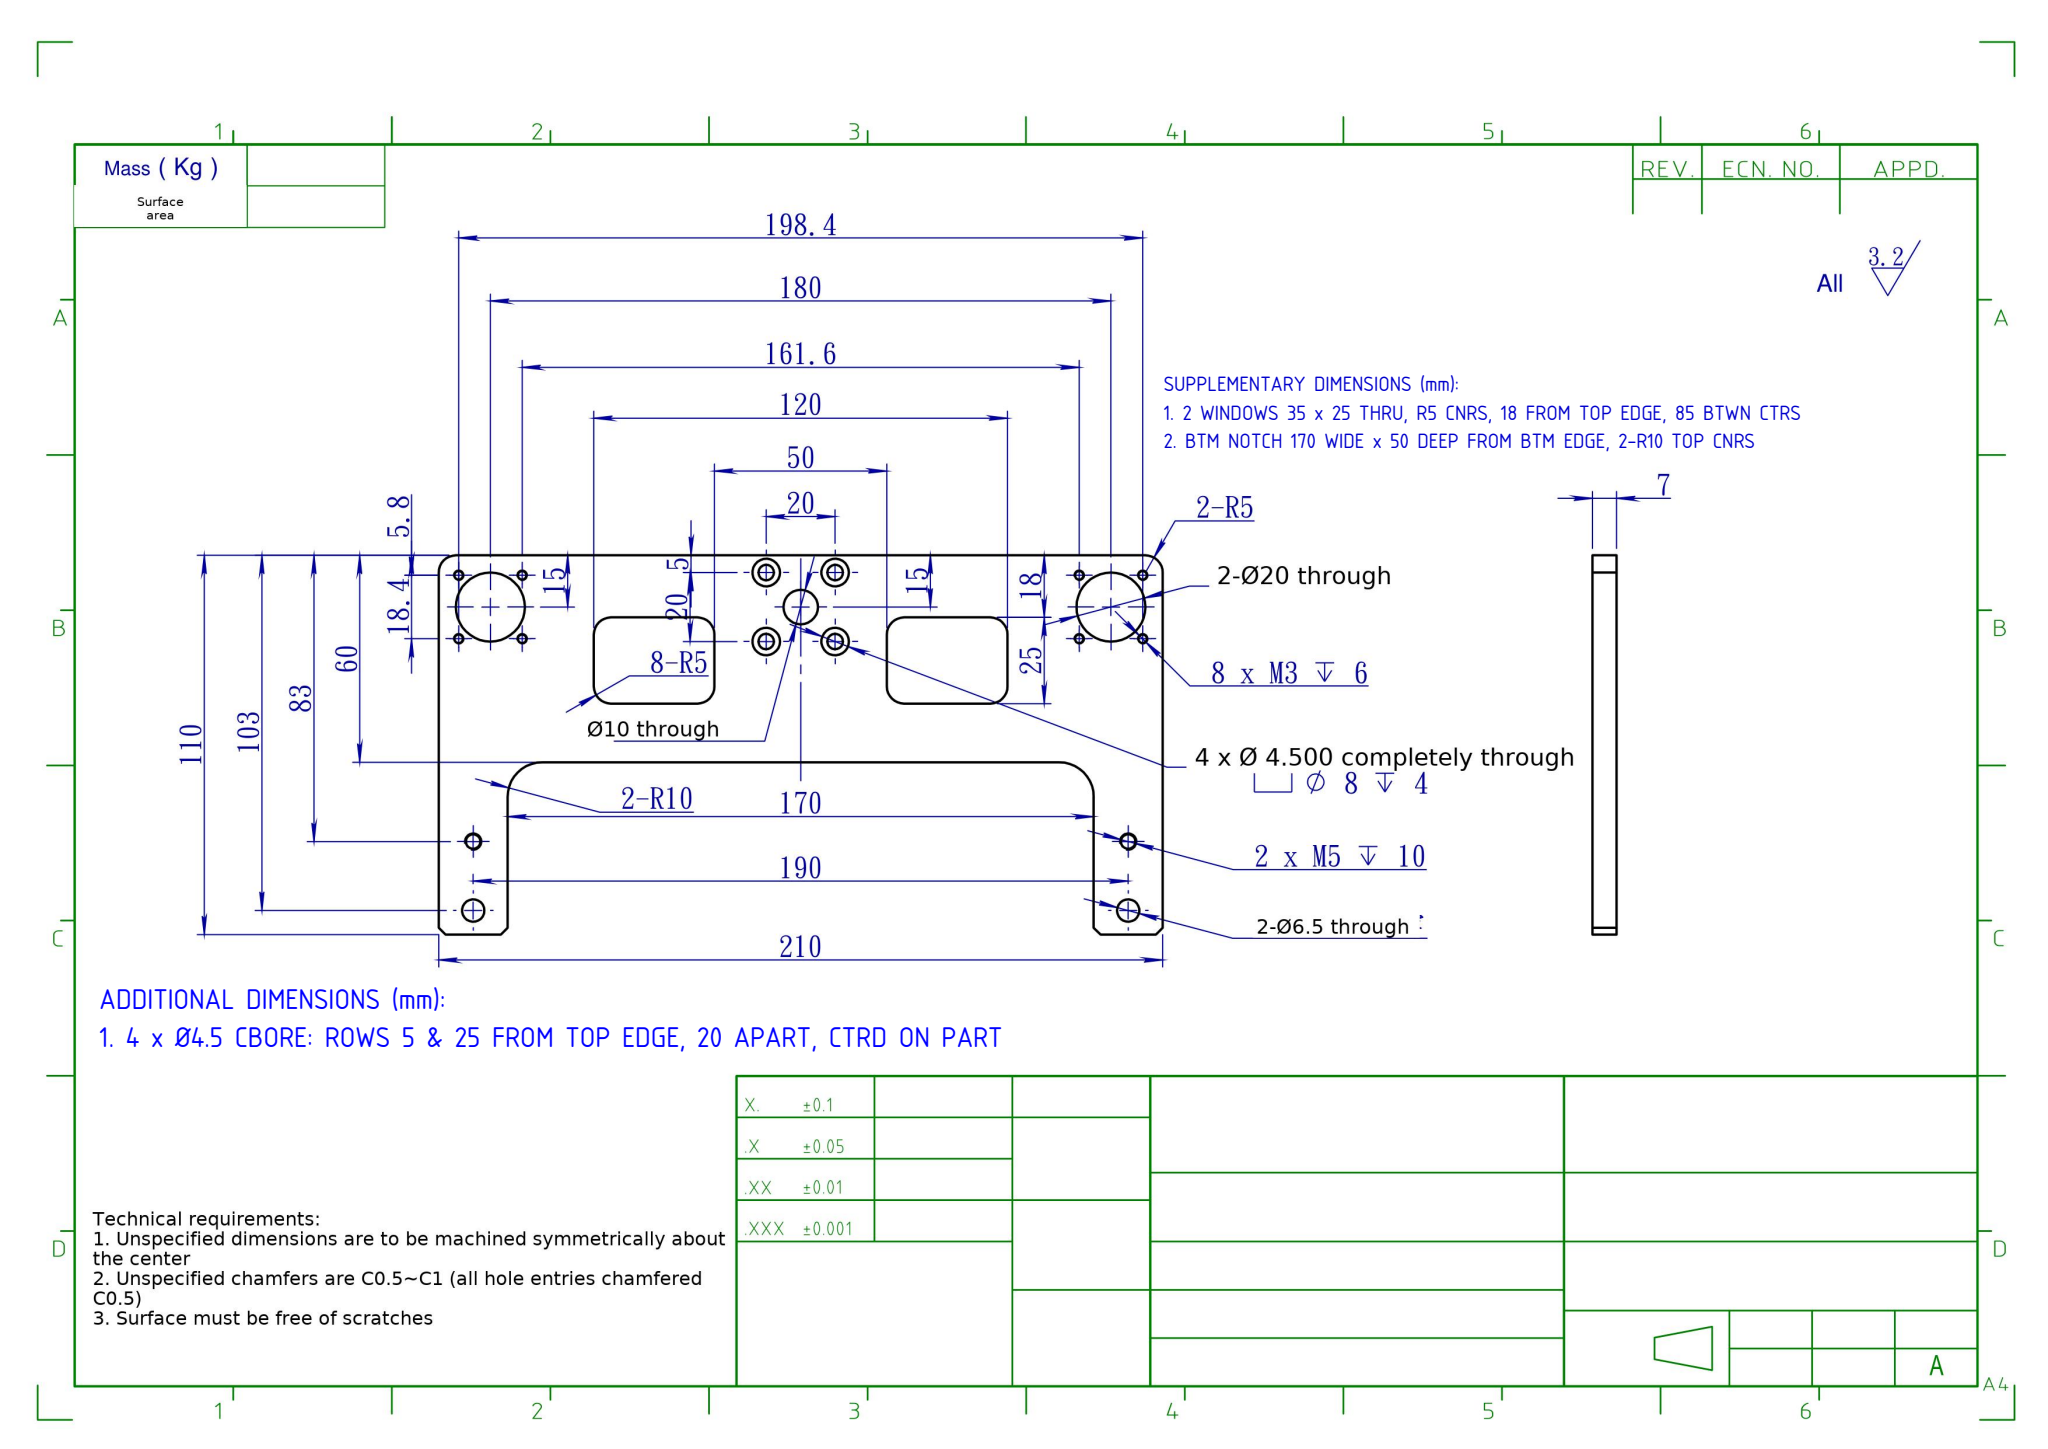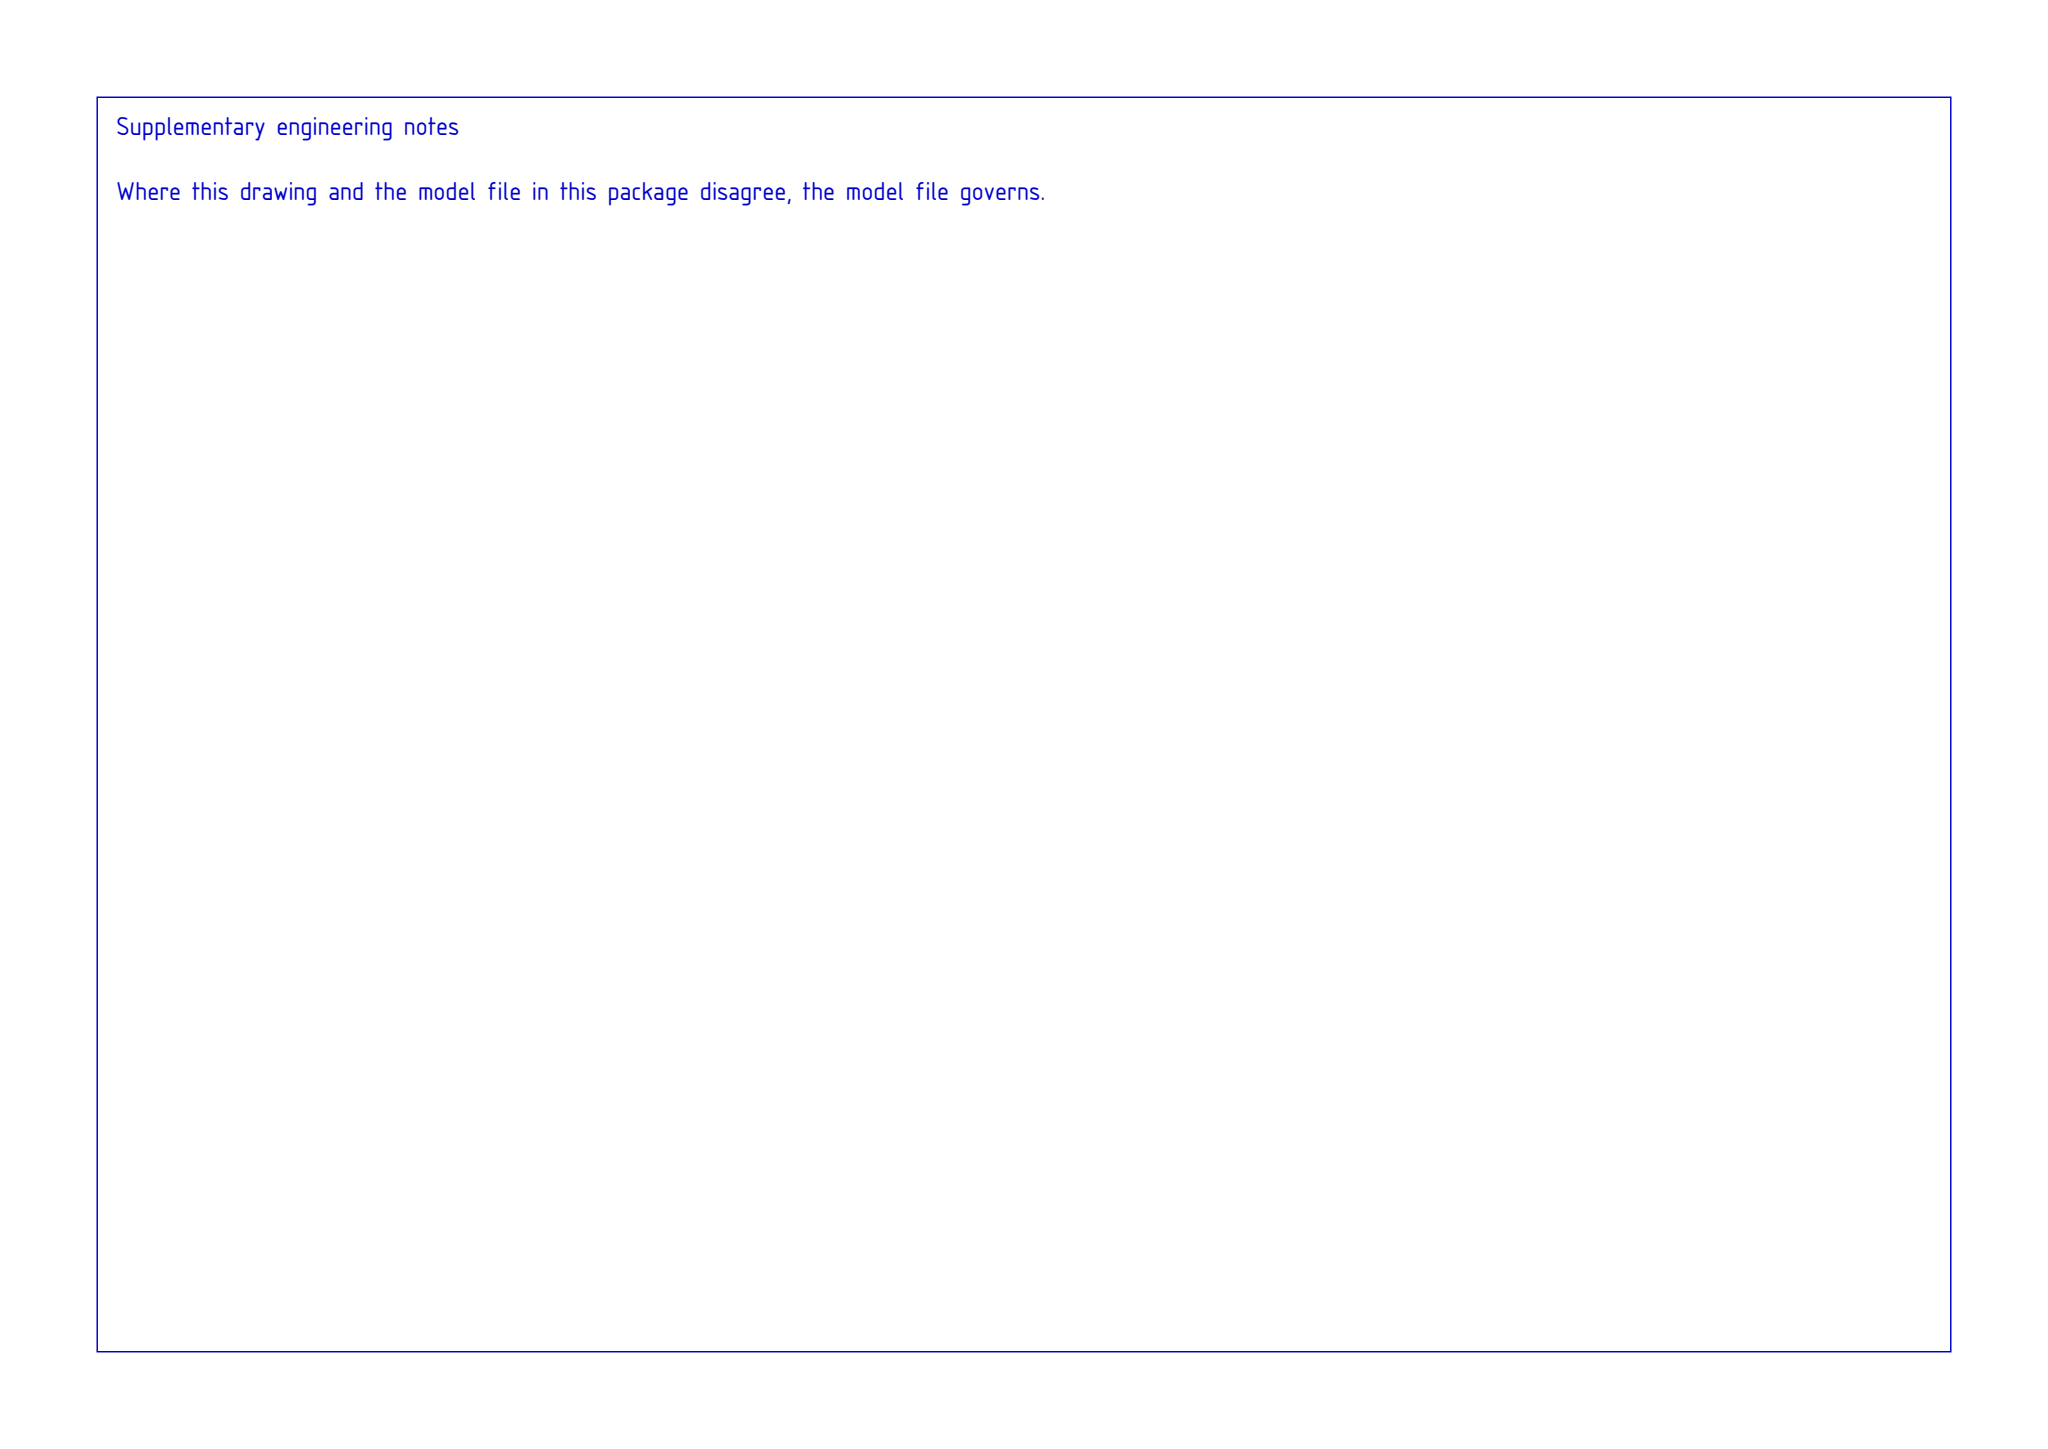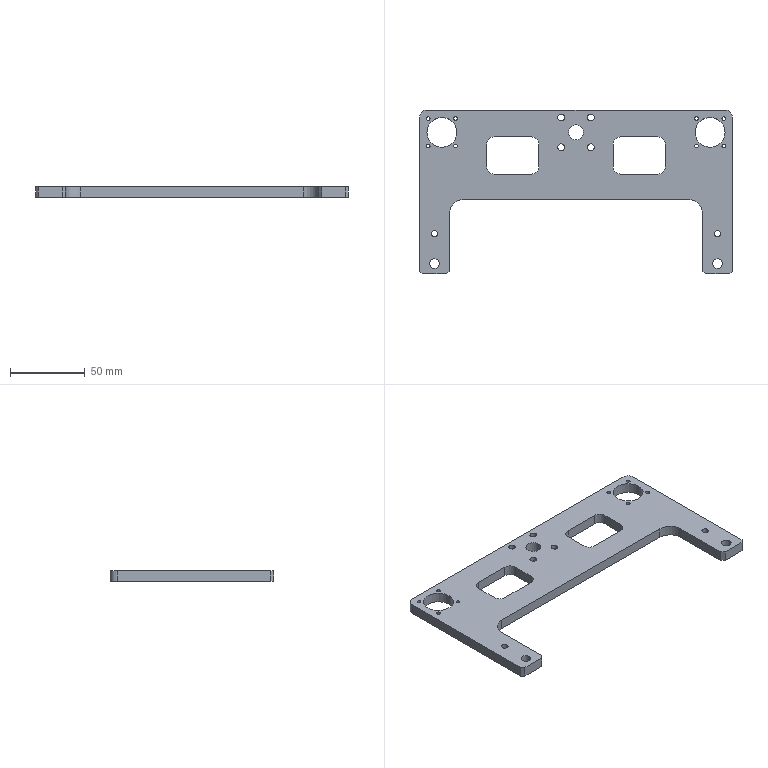Part | SolidWorks | mm | 1 solid | 84 faces | box 210 x 110 x 7 mm | volume 83543 mm3 | cylinder 58 | plane 26 | commonest cylinder face diameters 2.5 x16 10 x12 8 x8 4.5 x8 20 x6 4.2 x4 6.5 x4
build123d program:
from build123d import *

# Parameters (mm, degrees)
SKETCH1_2_W                                         = 210
SKETCH1_2_H                                         = 110
BOSS_EXTRUDE1_DEPTH                                 = 7
SKETCH2_2_W                                         = 170
SKETCH2_2_H                                         = 100
CUT_EXTRUDE1_2_DEPTH                                = 8
FILLET1_R                                           = 10
FILLET2_R                                           = 5
SKETCH3_2_R                                         = 5
SKETCH3_2_R_2                                       = 10
CUT_EXTRUDE2_2_DEPTH                                = 10
SKETCH1_R                                           = 3.25
CUT_EXTRUDE1_DEPTH                                  = 119.739
CHAMFER1_SIZE                                       = 2
M5_TAPPED_HOLE1_D                                   = 4.2
M5_TAPPED_HOLE1_DEPTH                               = 12.4
M5_TAPPED_HOLE1_TIP                                 = 1.262
M3_TAPPED_HOLE1_D                                   = 2.5
M3_TAPPED_HOLE1_DEPTH                               = 7.5
M3_TAPPED_HOLE1_TIP                                 = 0.7511
CBORE_FOR_M4_HEX_SOCKET_HEAD_CAP_SCREW1_D           = 4.5
CBORE_FOR_M4_HEX_SOCKET_HEAD_CAP_SCREW1_CBORE_D     = 8
CBORE_FOR_M4_HEX_SOCKET_HEAD_CAP_SCREW1_CBORE_DEPTH = 4
CUT_EXTRUDE2_DEPTH                                  = 119.739


with BuildPart() as part:
    # Sketch1_2 → Boss-Extrude1 (new body)
    with BuildSketch(Plane.XY):
        Rectangle(SKETCH1_2_W, SKETCH1_2_H)
    extrude(amount=BOSS_EXTRUDE1_DEPTH)

    # Sketch2_2 → Cut-Extrude1_2 (cut)
    with BuildSketch(Plane.XY.offset(7)):
        with Locations((0, -55)):
            Rectangle(SKETCH2_2_W, SKETCH2_2_H)
    extrude(amount=-CUT_EXTRUDE1_2_DEPTH, mode=Mode.SUBTRACT)

    # Fillet1
    fillet1_edges = [part.edges().sort_by_distance(p)[0] for p in [
        (-85, -5, 3.5),
        (85, -5, 3.5),
    ]]
    fillet(fillet1_edges, radius=FILLET1_R)

    # Fillet2
    fillet2_edges = [part.edges().sort_by_distance(p)[0] for p in [
        (-105, 55, 3.5),
        (105, 55, 3.5),
    ]]
    fillet(fillet2_edges, radius=FILLET2_R)

    # Sketch3_2 → Cut-Extrude2_2 (cut)
    with BuildSketch(Plane.XY.offset(7)):
        with Locations((0, 40)):
            Circle(SKETCH3_2_R)
        with Locations((-90, 40)):
            Circle(SKETCH3_2_R_2)
        with Locations((90, 40)):
            Circle(SKETCH3_2_R_2)
    extrude(amount=-CUT_EXTRUDE2_2_DEPTH, mode=Mode.SUBTRACT)

    # Sketch1 → Cut-Extrude1 (cut, through all)
    with BuildSketch(Plane.XY.offset(7)):
        with Locations((-95, -48)):
            Circle(SKETCH1_R)
        with Locations(Location((95, -48, 0), (0, 0, 180))):
            Circle(SKETCH1_R)
    extrude(amount=-CUT_EXTRUDE1_DEPTH, mode=Mode.SUBTRACT)

    # Chamfer1
    chamfer1_edges = [part.edges().sort_by_distance(p)[0] for p in [
        (-85, -55, 3.5),
        (85, -55, 3.5),
        (105, -55, 3.5),
        (-105, -55, 3.5),
    ]]
    chamfer(chamfer1_edges, length=CHAMFER1_SIZE)

    # M5 Tapped Hole1
    with Locations(Plane.XY.offset(7)):
        with Locations((-95, -28), (95, -28)):
            Hole(M5_TAPPED_HOLE1_D / 2, depth=M5_TAPPED_HOLE1_DEPTH)
            with Locations((0, 0, -(M5_TAPPED_HOLE1_DEPTH + M5_TAPPED_HOLE1_TIP / 2))):  # 118° drill point
                Cone(0, M5_TAPPED_HOLE1_D / 2, M5_TAPPED_HOLE1_TIP, mode=Mode.SUBTRACT)

    # M3 Tapped Hole1
    with Locations(Plane(origin=(0, 0, 0), x_dir=(-1, 0, 0), z_dir=(0, 0, -1))):
        with Locations((99.2, 49.2), (99.2, 30.8), (80.8, 30.8), (80.8, 49.2), (-80.8, 49.2), (-80.8, 30.8), (-99.2, 30.8), (-99.2, 49.2)):
            Hole(M3_TAPPED_HOLE1_D / 2, depth=M3_TAPPED_HOLE1_DEPTH)
            with Locations((0, 0, -(M3_TAPPED_HOLE1_DEPTH + M3_TAPPED_HOLE1_TIP / 2))):  # 118° drill point
                Cone(0, M3_TAPPED_HOLE1_D / 2, M3_TAPPED_HOLE1_TIP, mode=Mode.SUBTRACT)

    # CBORE for M4 Hex Socket Head Cap Screw1 (through all)
    with Locations(Plane(origin=(0, 0, 0), x_dir=(-1, 0, 0), z_dir=(0, 0, -1))):
        with Locations((-10, 50), (-10, 30), (10, 30), (10, 50)):
            CounterBoreHole(CBORE_FOR_M4_HEX_SOCKET_HEAD_CAP_SCREW1_D / 2, CBORE_FOR_M4_HEX_SOCKET_HEAD_CAP_SCREW1_CBORE_D / 2, CBORE_FOR_M4_HEX_SOCKET_HEAD_CAP_SCREW1_CBORE_DEPTH)

    # Sketch12 → Cut-Extrude2 (cut, through all)
    with BuildSketch(Plane.XY.offset(7)):
        with BuildLine():
            Line((-55, 37), (-30, 37))
            ThreePointArc((-30, 37), (-26.464, 35.536), (-25, 32))
            Line((-25, 32), (-25, 17))
            ThreePointArc((-25, 17), (-26.464, 13.464), (-30, 12))
            Line((-30, 12), (-55, 12))
            ThreePointArc((-55, 12), (-58.536, 13.464), (-60, 17))
            Line((-60, 17), (-60, 32))
            ThreePointArc((-60, 32), (-58.536, 35.536), (-55, 37))
        make_face()
        with BuildLine():
            Line((25, 32), (25, 17))
            ThreePointArc((25, 17), (26.464, 13.464), (30, 12))
            Line((30, 12), (55, 12))
            ThreePointArc((55, 12), (58.536, 13.464), (60, 17))
            Line((60, 17), (60, 32))
            ThreePointArc((60, 32), (58.536, 35.536), (55, 37))
            Line((55, 37), (30, 37))
            ThreePointArc((30, 37), (26.464, 35.536), (25, 32))
        make_face()
    extrude(amount=-CUT_EXTRUDE2_DEPTH, mode=Mode.SUBTRACT)


solid = part.part